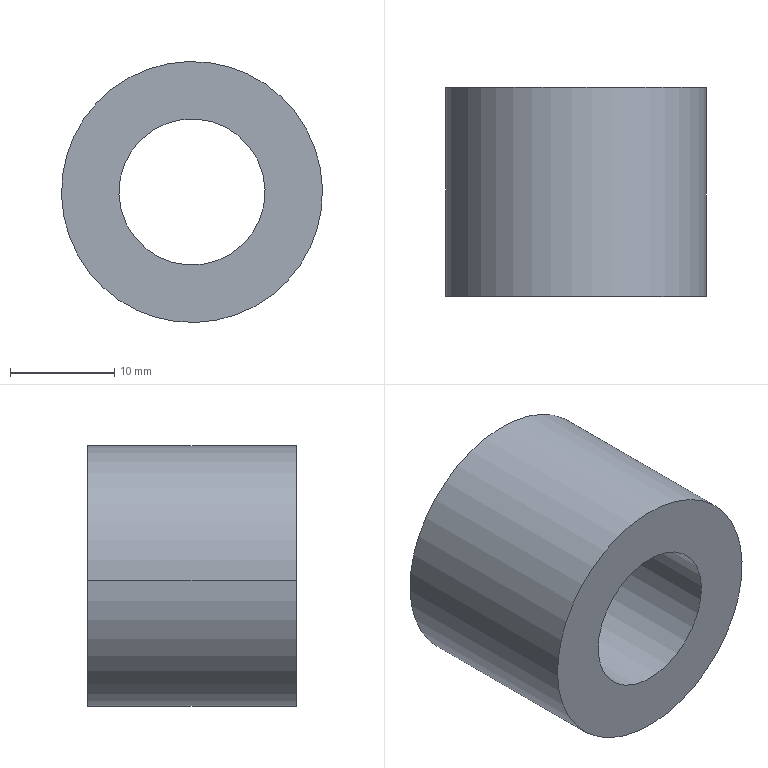Component | SolidWorks | LowerBushing-1 | 1 solid | 6 faces | box 25 x 20 x 25 mm | volume 6739 mm3 | cylinder 4 | plane 2 | commonest cylinder face diameters 14 x2 25 x2
build123d program:
from build123d import *

# Parameters (mm, degrees)
SKETCH1_R           = 12.5
SKETCH1_R_2         = 7
BOSS_EXTRUDE1_DEPTH = 20


with BuildPart() as part:
    # Sketch1 → Boss-Extrude1 (new body)
    with BuildSketch(Plane.XY):
        with Locations((-75, 62.5)):
            Circle(SKETCH1_R)
        with Locations((-75, 62.5)):
            Circle(SKETCH1_R_2, mode=Mode.SUBTRACT)
    extrude(amount=BOSS_EXTRUDE1_DEPTH)


solid = part.part

# Placed as in the assembly
solid = solid.moved(Location((0, 150.512, -125), (90, 0, 0)))
STEP:
#1=CARTESIAN_POINT('',(-3.228,5.926,-2.47));
#2=VERTEX_POINT('',#1);
#3=CARTESIAN_POINT('',(-2.677,5.926,-2.452));
#4=VERTEX_POINT('',#3);
#5=CARTESIAN_POINT('',(-2.953,5.926,-2.461));
#6=DIRECTION('',(0.,1.,0.));
#7=DIRECTION('',(0.9995,0.,0.03311));
#8=AXIS2_PLACEMENT_3D('',#5,#6,#7);
#9=CIRCLE('',#8,0.2756);
#10=EDGE_CURVE('',#2,#4,#9,.T.);
#11=ORIENTED_EDGE('',*,*,#10,.T.);
#12=CARTESIAN_POINT('',(-2.677,5.138,-2.452));
#13=VERTEX_POINT('',#12);
#14=CARTESIAN_POINT('',(-2.677,5.926,-2.452));
#15=DIRECTION('',(0.,-1.,0.));
#16=VECTOR('',#15,39.37);
#17=LINE('',#14,#16);
#18=EDGE_CURVE('',#4,#13,#17,.T.);
#19=ORIENTED_EDGE('',*,*,#18,.T.);
#20=CARTESIAN_POINT('',(-3.228,5.138,-2.47));
#21=VERTEX_POINT('',#20);
#22=CARTESIAN_POINT('',(-2.953,5.138,-2.461));
#23=DIRECTION('',(0.,1.,0.));
#24=DIRECTION('',(0.9995,0.,0.03311));
#25=AXIS2_PLACEMENT_3D('',#22,#23,#24);
#26=CIRCLE('',#25,0.2756);
#27=EDGE_CURVE('',#21,#13,#26,.T.);
#28=ORIENTED_EDGE('',*,*,#27,.F.);
#29=CARTESIAN_POINT('',(-3.228,5.926,-2.47));
#30=DIRECTION('',(0.,-1.,0.));
#31=VECTOR('',#30,39.37);
#32=LINE('',#29,#31);
#33=EDGE_CURVE('',#2,#21,#32,.T.);
#34=ORIENTED_EDGE('',*,*,#33,.F.);
#35=EDGE_LOOP('',(#11,#19,#28,#34));
#36=FACE_OUTER_BOUND('',#35,.T.);
#37=CARTESIAN_POINT('',(-2.953,5.926,-2.461));
#38=DIRECTION('',(0.,-1.,0.));
#39=DIRECTION('',(-0.9995,0.,-0.03311));
#40=AXIS2_PLACEMENT_3D('',#37,#38,#39);
#41=CYLINDRICAL_SURFACE('',#40,0.2756);
#42=ADVANCED_FACE('',(#36),#41,.F.);
#43=CARTESIAN_POINT('',(-2.461,5.926,-2.444));
#44=VERTEX_POINT('',#43);
#45=CARTESIAN_POINT('',(-3.445,5.926,-2.477));
#46=VERTEX_POINT('',#45);
#47=CARTESIAN_POINT('',(-2.953,5.926,-2.461));
#48=DIRECTION('',(0.,1.,0.));
#49=DIRECTION('',(0.9995,0.,0.03311));
#50=AXIS2_PLACEMENT_3D('',#47,#48,#49);
#51=CIRCLE('',#50,0.4921);
#52=EDGE_CURVE('',#44,#46,#51,.T.);
#53=ORIENTED_EDGE('',*,*,#52,.F.);
#54=CARTESIAN_POINT('',(-2.461,5.138,-2.444));
#55=VERTEX_POINT('',#54);
#56=CARTESIAN_POINT('',(-2.461,5.926,-2.444));
#57=DIRECTION('',(0.,-1.,0.));
#58=VECTOR('',#57,39.37);
#59=LINE('',#56,#58);
#60=EDGE_CURVE('',#44,#55,#59,.T.);
#61=ORIENTED_EDGE('',*,*,#60,.T.);
#62=CARTESIAN_POINT('',(-3.445,5.138,-2.477));
#63=VERTEX_POINT('',#62);
#64=CARTESIAN_POINT('',(-2.953,5.138,-2.461));
#65=DIRECTION('',(0.,1.,0.));
#66=DIRECTION('',(0.9995,0.,0.03311));
#67=AXIS2_PLACEMENT_3D('',#64,#65,#66);
#68=CIRCLE('',#67,0.4921);
#69=EDGE_CURVE('',#55,#63,#68,.T.);
#70=ORIENTED_EDGE('',*,*,#69,.T.);
#71=CARTESIAN_POINT('',(-3.445,5.926,-2.477));
#72=DIRECTION('',(0.,-1.,0.));
#73=VECTOR('',#72,39.37);
#74=LINE('',#71,#73);
#75=EDGE_CURVE('',#46,#63,#74,.T.);
#76=ORIENTED_EDGE('',*,*,#75,.F.);
#77=EDGE_LOOP('',(#53,#61,#70,#76));
#78=FACE_OUTER_BOUND('',#77,.T.);
#79=CARTESIAN_POINT('',(-2.953,5.926,-2.461));
#80=DIRECTION('',(0.,-1.,0.));
#81=DIRECTION('',(-0.9995,0.,-0.03311));
#82=AXIS2_PLACEMENT_3D('',#79,#80,#81);
#83=CYLINDRICAL_SURFACE('',#82,0.4921);
#84=ADVANCED_FACE('',(#78),#83,.T.);
#85=CARTESIAN_POINT('',(-2.953,5.926,-2.461));
#86=DIRECTION('',(0.,1.,0.));
#87=DIRECTION('',(0.9995,0.,0.03311));
#88=AXIS2_PLACEMENT_3D('',#85,#86,#87);
#89=CIRCLE('',#88,0.4921);
#90=EDGE_CURVE('',#46,#44,#89,.T.);
#91=ORIENTED_EDGE('',*,*,#90,.T.);
#92=ORIENTED_EDGE('',*,*,#52,.T.);
#93=EDGE_LOOP('',(#91,#92));
#94=FACE_OUTER_BOUND('',#93,.T.);
#95=ORIENTED_EDGE('',*,*,#10,.F.);
#96=CARTESIAN_POINT('',(-2.953,5.926,-2.461));
#97=DIRECTION('',(0.,1.,0.));
#98=DIRECTION('',(0.9995,0.,0.03311));
#99=AXIS2_PLACEMENT_3D('',#96,#97,#98);
#100=CIRCLE('',#99,0.2756);
#101=EDGE_CURVE('',#4,#2,#100,.T.);
#102=ORIENTED_EDGE('',*,*,#101,.F.);
#103=EDGE_LOOP('',(#95,#102));
#104=FACE_BOUND('',#103,.T.);
#105=CARTESIAN_POINT('',(-2.953,5.926,-2.461));
#106=DIRECTION('',(0.,1.,0.));
#107=DIRECTION('',(0.9995,0.,0.03311));
#108=AXIS2_PLACEMENT_3D('',#105,#106,#107);
#109=PLANE('',#108);
#110=ADVANCED_FACE('',(#94,#104),#109,.T.);
#111=CARTESIAN_POINT('',(-2.953,5.138,-2.461));
#112=DIRECTION('',(0.,1.,0.));
#113=DIRECTION('',(0.9995,0.,0.03311));
#114=AXIS2_PLACEMENT_3D('',#111,#112,#113);
#115=CIRCLE('',#114,0.4921);
#116=EDGE_CURVE('',#63,#55,#115,.T.);
#117=ORIENTED_EDGE('',*,*,#116,.F.);
#118=ORIENTED_EDGE('',*,*,#69,.F.);
#119=EDGE_LOOP('',(#117,#118));
#120=FACE_OUTER_BOUND('',#119,.T.);
#121=ORIENTED_EDGE('',*,*,#27,.T.);
#122=CARTESIAN_POINT('',(-2.953,5.138,-2.461));
#123=DIRECTION('',(0.,1.,0.));
#124=DIRECTION('',(0.9995,0.,0.03311));
#125=AXIS2_PLACEMENT_3D('',#122,#123,#124);
#126=CIRCLE('',#125,0.2756);
#127=EDGE_CURVE('',#13,#21,#126,.T.);
#128=ORIENTED_EDGE('',*,*,#127,.T.);
#129=EDGE_LOOP('',(#121,#128));
#130=FACE_BOUND('',#129,.T.);
#131=CARTESIAN_POINT('',(-2.953,5.138,-2.461));
#132=DIRECTION('',(0.,1.,0.));
#133=DIRECTION('',(0.9995,0.,0.03311));
#134=AXIS2_PLACEMENT_3D('',#131,#132,#133);
#135=PLANE('',#134);
#136=ADVANCED_FACE('',(#120,#130),#135,.F.);
#137=ORIENTED_EDGE('',*,*,#60,.F.);
#138=ORIENTED_EDGE('',*,*,#90,.F.);
#139=ORIENTED_EDGE('',*,*,#75,.T.);
#140=ORIENTED_EDGE('',*,*,#116,.T.);
#141=EDGE_LOOP('',(#137,#138,#139,#140));
#142=FACE_OUTER_BOUND('',#141,.T.);
#143=CARTESIAN_POINT('',(-2.953,5.926,-2.461));
#144=DIRECTION('',(0.,-1.,0.));
#145=DIRECTION('',(-0.9995,0.,-0.03311));
#146=AXIS2_PLACEMENT_3D('',#143,#144,#145);
#147=CYLINDRICAL_SURFACE('',#146,0.4921);
#148=ADVANCED_FACE('',(#142),#147,.T.);
#149=ORIENTED_EDGE('',*,*,#18,.F.);
#150=ORIENTED_EDGE('',*,*,#101,.T.);
#151=ORIENTED_EDGE('',*,*,#33,.T.);
#152=ORIENTED_EDGE('',*,*,#127,.F.);
#153=EDGE_LOOP('',(#149,#150,#151,#152));
#154=FACE_OUTER_BOUND('',#153,.T.);
#155=CARTESIAN_POINT('',(-2.953,5.926,-2.461));
#156=DIRECTION('',(0.,-1.,0.));
#157=DIRECTION('',(-0.9995,0.,-0.03311));
#158=AXIS2_PLACEMENT_3D('',#155,#156,#157);
#159=CYLINDRICAL_SURFACE('',#158,0.2756);
#160=ADVANCED_FACE('',(#154),#159,.F.);
#161=CLOSED_SHELL('',(#42,#84,#110,#136,#148,#160));
#162=MANIFOLD_SOLID_BREP('',#161);
#163=CARTESIAN_POINT('',(0.,0.,0.));
#164=DIRECTION('',(0.,0.,1.));
#165=DIRECTION('',(1.,0.,0.));
#166=AXIS2_PLACEMENT_3D('',#163,#164,#165);
#167=(LENGTH_UNIT()NAMED_UNIT(*)SI_UNIT($,.METRE.));
#168=LENGTH_MEASURE_WITH_UNIT(LENGTH_MEASURE(0.0254),#167);
#169=DIMENSIONAL_EXPONENTS(1.,0.,0.,0.,0.,0.,0.);
#170=(CONVERSION_BASED_UNIT('',#168)LENGTH_UNIT()NAMED_UNIT(#169));
#171=UNCERTAINTY_MEASURE_WITH_UNIT(LENGTH_MEASURE(0.00001),#170,'','');
#172=(NAMED_UNIT(*)PLANE_ANGLE_UNIT()SI_UNIT($,.RADIAN.));
#173=(NAMED_UNIT(*)SI_UNIT($,.STERADIAN.)SOLID_ANGLE_UNIT());
#174=(GEOMETRIC_REPRESENTATION_CONTEXT(3)GLOBAL_UNCERTAINTY_ASSIGNED_CONTEXT((#171))GLOBAL_UNIT_ASSIGNED_CONTEXT((#170,#172,#173))REPRESENTATION_CONTEXT('',''));
#175=ADVANCED_BREP_SHAPE_REPRESENTATION('',(#162,#166),#174);
#176=COLOUR_RGB('',0.7922,0.8196,0.9333);
#177=FILL_AREA_STYLE_COLOUR('',#176);
#178=FILL_AREA_STYLE('',(#177));
#179=SURFACE_STYLE_FILL_AREA(#178);
#180=SURFACE_SIDE_STYLE('',(#179));
#181=SURFACE_STYLE_USAGE(.BOTH.,#180);
#182=PRESENTATION_STYLE_ASSIGNMENT((#181));
#183=STYLED_ITEM('',(#182),#162);
#184=PRESENTATION_LAYER_ASSIGNMENT('','',(#183));
#185=(LENGTH_UNIT()NAMED_UNIT(*)SI_UNIT($,.METRE.));
#186=LENGTH_MEASURE_WITH_UNIT(LENGTH_MEASURE(0.0254),#185);
#187=DIMENSIONAL_EXPONENTS(1.,0.,0.,0.,0.,0.,0.);
#188=(CONVERSION_BASED_UNIT('',#186)LENGTH_UNIT()NAMED_UNIT(#187));
#189=UNCERTAINTY_MEASURE_WITH_UNIT(LENGTH_MEASURE(0.00001),#188,'','');
#190=(NAMED_UNIT(*)PLANE_ANGLE_UNIT()SI_UNIT($,.RADIAN.));
#191=(NAMED_UNIT(*)SI_UNIT($,.STERADIAN.)SOLID_ANGLE_UNIT());
#192=(GEOMETRIC_REPRESENTATION_CONTEXT(3)GLOBAL_UNCERTAINTY_ASSIGNED_CONTEXT((#189))GLOBAL_UNIT_ASSIGNED_CONTEXT((#188,#190,#191))REPRESENTATION_CONTEXT('',''));
#193=MECHANICAL_DESIGN_GEOMETRIC_PRESENTATION_REPRESENTATION('',(#183),#192);